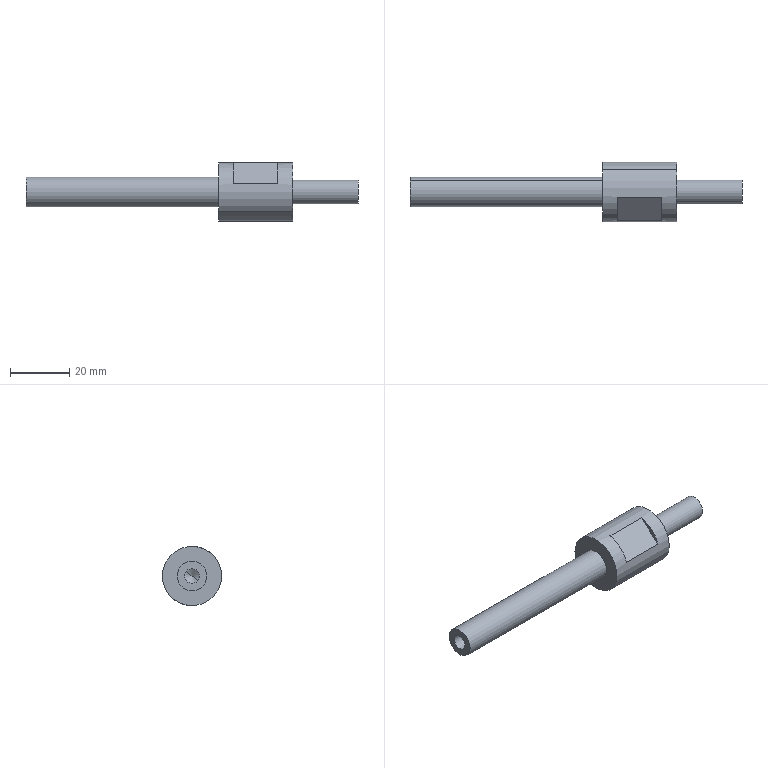Component | SolidWorks | ElectricalBoxAssembly2-1_RollerAxis-1 | 1 solid | 20 faces | box 112 x 20 x 20 mm | volume 13341 mm3 | plane 10 | cylinder 8 | cone 2 | commonest cylinder face diameters 5 x2 10 x2 20 x2 8 x2
build123d program:
from build123d import *

# Parameters (mm, degrees)
CUT_EXTRUDE1_DEPTH      = 113.889
CUT_EXTRUDE1_DEPTH_BACK = 113.889
SKETCH2_W               = 15
SKETCH2_H               = 1.5
M6_TAPPED_HOLE1_D       = 5
M6_TAPPED_HOLE1_DEPTH   = 20
M6_TAPPED_HOLE1_TIP     = 1.502


with BuildPart() as part:
    # Sketch1 → Revolve1 (revolve)
    with BuildSketch(Plane.XY, mode=Mode.PRIVATE) as revolve1_sk:
        Polygon((0, 0), (112, 0), (112, 5), (47, 5), (47, 10), (22, 10), (22, 4), (0, 4), align=None)
    revolve(revolve1_sk.sketch.rotate(Axis((0, 0, 0), (1, 0, 0)), 90), axis=Axis((0, 0, 0), (1, 0, 0)))

    # Sketch2 → Cut-Extrude1 (cut, two sides: drawn at the far end of the back side and taken through both)
    with BuildSketch(Plane.XY.offset(-CUT_EXTRUDE1_DEPTH_BACK)):
        with Locations((34.5, 9.25)):
            Rectangle(SKETCH2_W, SKETCH2_H)
        with Locations((34.5, -9.25)):
            Rectangle(SKETCH2_W, SKETCH2_H)
    extrude(amount=CUT_EXTRUDE1_DEPTH + CUT_EXTRUDE1_DEPTH_BACK, mode=Mode.SUBTRACT)

    # M6 Tapped Hole1
    with Locations(Plane(origin=(112, 0, 0), x_dir=(0, 0, -1), z_dir=(1, 0, 0))):
        with Locations((0, 0)):
            Hole(M6_TAPPED_HOLE1_D / 2, depth=M6_TAPPED_HOLE1_DEPTH)
            with Locations((0, 0, -(M6_TAPPED_HOLE1_DEPTH + M6_TAPPED_HOLE1_TIP / 2))):  # 118° drill point
                Cone(0, M6_TAPPED_HOLE1_D / 2, M6_TAPPED_HOLE1_TIP, mode=Mode.SUBTRACT)


solid = part.part

# Placed as in the assembly
solid = solid.moved(Location((765.468, -65.334, 1576.399), (-48.376, 0, 180)))
STEP:
#1=COLOUR_RGB('',0.7922,0.8196,0.9333);
#2=FILL_AREA_STYLE_COLOUR('',#1);
#3=FILL_AREA_STYLE('',(#2));
#4=SURFACE_STYLE_FILL_AREA(#3);
#5=SURFACE_SIDE_STYLE('',(#4));
#6=SURFACE_STYLE_USAGE(.BOTH.,#5);
#7=PRESENTATION_STYLE_ASSIGNMENT((#6));
#8=CARTESIAN_POINT('',(26.514,-2.499,62.128));
#9=VERTEX_POINT('',#8);
#10=CARTESIAN_POINT('',(26.514,-2.646,61.998));
#11=VERTEX_POINT('',#10);
#12=CARTESIAN_POINT('',(26.514,-2.572,62.063));
#13=DIRECTION('',(-1.,0.,-0.));
#14=DIRECTION('',(0.,-0.7475,-0.6642));
#15=AXIS2_PLACEMENT_3D('',#12,#13,#14);
#16=CIRCLE('',#15,0.09843);
#17=EDGE_CURVE('',#9,#11,#16,.T.);
#18=ORIENTED_EDGE('',*,*,#17,.F.);
#19=CARTESIAN_POINT('',(25.727,-2.499,62.128));
#20=VERTEX_POINT('',#19);
#21=CARTESIAN_POINT('',(25.727,-2.499,62.128));
#22=DIRECTION('',(-1.,0.,-0.));
#23=VECTOR('',#22,39.37);
#24=LINE('',#21,#23);
#25=EDGE_CURVE('',#9,#20,#24,.T.);
#26=ORIENTED_EDGE('',*,*,#25,.T.);
#27=CARTESIAN_POINT('',(25.727,-2.646,61.998));
#28=VERTEX_POINT('',#27);
#29=CARTESIAN_POINT('',(25.727,-2.572,62.063));
#30=DIRECTION('',(-1.,0.,-0.));
#31=DIRECTION('',(0.,-0.7475,-0.6642));
#32=AXIS2_PLACEMENT_3D('',#29,#30,#31);
#33=CIRCLE('',#32,0.09843);
#34=EDGE_CURVE('',#20,#28,#33,.T.);
#35=ORIENTED_EDGE('',*,*,#34,.T.);
#36=CARTESIAN_POINT('',(25.727,-2.646,61.998));
#37=DIRECTION('',(-1.,0.,-0.));
#38=VECTOR('',#37,39.37);
#39=LINE('',#36,#38);
#40=EDGE_CURVE('',#11,#28,#39,.T.);
#41=ORIENTED_EDGE('',*,*,#40,.F.);
#42=EDGE_LOOP('',(#18,#26,#35,#41));
#43=FACE_OUTER_BOUND('',#42,.T.);
#44=CARTESIAN_POINT('',(25.727,-2.572,62.063));
#45=DIRECTION('',(-1.,0.,-0.));
#46=DIRECTION('',(0.,-0.7475,-0.6642));
#47=AXIS2_PLACEMENT_3D('',#44,#45,#46);
#48=CYLINDRICAL_SURFACE('',#47,0.09843);
#49=ADVANCED_FACE('',(#43),#48,.F.);
#50=CARTESIAN_POINT('',(26.574,-2.572,62.063));
#51=VERTEX_POINT('',#50);
#52=CARTESIAN_POINT('',(26.514,-2.646,61.998));
#53=DIRECTION('',(-0.515,-0.6408,-0.5694));
#54=VECTOR('',#53,39.37);
#55=LINE('',#52,#54);
#56=EDGE_CURVE('',#51,#11,#55,.T.);
#57=ORIENTED_EDGE('',*,*,#56,.F.);
#58=CARTESIAN_POINT('',(26.514,-2.499,62.128));
#59=DIRECTION('',(-0.515,0.6408,0.5694));
#60=VECTOR('',#59,39.37);
#61=LINE('',#58,#60);
#62=EDGE_CURVE('',#51,#9,#61,.T.);
#63=ORIENTED_EDGE('',*,*,#62,.T.);
#64=ORIENTED_EDGE('',*,*,#17,.T.);
#65=EDGE_LOOP('',(#57,#63,#64));
#66=FACE_OUTER_BOUND('',#65,.T.);
#67=CARTESIAN_POINT('',(26.514,-2.572,62.063));
#68=DIRECTION('',(-1.,0.,-0.));
#69=DIRECTION('',(0.,-0.7475,-0.6642));
#70=AXIS2_PLACEMENT_3D('',#67,#68,#69);
#71=CONICAL_SURFACE('',#70,0.09843,1.03);
#72=ADVANCED_FACE('',(#66),#71,.F.);
#73=CARTESIAN_POINT('',(25.727,-2.425,62.194));
#74=VERTEX_POINT('',#73);
#75=CARTESIAN_POINT('',(25.727,-2.719,61.932));
#76=VERTEX_POINT('',#75);
#77=CARTESIAN_POINT('',(25.727,-2.572,62.063));
#78=DIRECTION('',(1.,-0.,0.));
#79=DIRECTION('',(0.,0.7475,0.6642));
#80=AXIS2_PLACEMENT_3D('',#77,#78,#79);
#81=CIRCLE('',#80,0.1969);
#82=EDGE_CURVE('',#74,#76,#81,.T.);
#83=ORIENTED_EDGE('',*,*,#82,.T.);
#84=CARTESIAN_POINT('',(28.286,-2.719,61.932));
#85=VERTEX_POINT('',#84);
#86=CARTESIAN_POINT('',(30.137,-2.719,61.932));
#87=DIRECTION('',(1.,-0.,0.));
#88=VECTOR('',#87,39.37);
#89=LINE('',#86,#88);
#90=EDGE_CURVE('',#76,#85,#89,.T.);
#91=ORIENTED_EDGE('',*,*,#90,.T.);
#92=CARTESIAN_POINT('',(28.286,-2.425,62.194));
#93=VERTEX_POINT('',#92);
#94=CARTESIAN_POINT('',(28.286,-2.572,62.063));
#95=DIRECTION('',(1.,-0.,0.));
#96=DIRECTION('',(0.,0.7475,0.6642));
#97=AXIS2_PLACEMENT_3D('',#94,#95,#96);
#98=CIRCLE('',#97,0.1969);
#99=EDGE_CURVE('',#93,#85,#98,.T.);
#100=ORIENTED_EDGE('',*,*,#99,.F.);
#101=CARTESIAN_POINT('',(30.137,-2.425,62.194));
#102=DIRECTION('',(1.,-0.,0.));
#103=VECTOR('',#102,39.37);
#104=LINE('',#101,#103);
#105=EDGE_CURVE('',#74,#93,#104,.T.);
#106=ORIENTED_EDGE('',*,*,#105,.F.);
#107=EDGE_LOOP('',(#83,#91,#100,#106));
#108=FACE_OUTER_BOUND('',#107,.T.);
#109=CARTESIAN_POINT('',(30.137,-2.572,62.063));
#110=DIRECTION('',(1.,-0.,0.));
#111=DIRECTION('',(0.,0.7475,0.6642));
#112=AXIS2_PLACEMENT_3D('',#109,#110,#111);
#113=CYLINDRICAL_SURFACE('',#112,0.1969);
#114=ADVANCED_FACE('',(#108),#113,.T.);
#115=CARTESIAN_POINT('',(28.483,-2.95,62.175));
#116=VERTEX_POINT('',#115);
#117=CARTESIAN_POINT('',(28.483,-2.639,62.451));
#118=VERTEX_POINT('',#117);
#119=CARTESIAN_POINT('',(28.483,-2.572,62.063));
#120=DIRECTION('',(-1.,-0.,0.));
#121=DIRECTION('',(0.,-0.6642,0.7475));
#122=AXIS2_PLACEMENT_3D('',#119,#120,#121);
#123=CIRCLE('',#122,0.3937);
#124=EDGE_CURVE('',#116,#118,#123,.T.);
#125=ORIENTED_EDGE('',*,*,#124,.T.);
#126=CARTESIAN_POINT('',(29.074,-2.639,62.451));
#127=VERTEX_POINT('',#126);
#128=CARTESIAN_POINT('',(30.137,-2.639,62.451));
#129=DIRECTION('',(1.,-0.,0.));
#130=VECTOR('',#129,39.37);
#131=LINE('',#128,#130);
#132=EDGE_CURVE('',#118,#127,#131,.T.);
#133=ORIENTED_EDGE('',*,*,#132,.T.);
#134=CARTESIAN_POINT('',(29.074,-2.95,62.175));
#135=VERTEX_POINT('',#134);
#136=CARTESIAN_POINT('',(29.074,-2.572,62.063));
#137=DIRECTION('',(1.,-0.,0.));
#138=DIRECTION('',(0.,0.7475,0.6642));
#139=AXIS2_PLACEMENT_3D('',#136,#137,#138);
#140=CIRCLE('',#139,0.3937);
#141=EDGE_CURVE('',#127,#135,#140,.T.);
#142=ORIENTED_EDGE('',*,*,#141,.T.);
#143=CARTESIAN_POINT('',(30.137,-2.95,62.175));
#144=DIRECTION('',(-1.,0.,-0.));
#145=VECTOR('',#144,39.37);
#146=LINE('',#143,#145);
#147=EDGE_CURVE('',#135,#116,#146,.T.);
#148=ORIENTED_EDGE('',*,*,#147,.T.);
#149=EDGE_LOOP('',(#125,#133,#142,#148));
#150=FACE_BOUND('',#149,.T.);
#151=CARTESIAN_POINT('',(28.286,-2.278,62.324));
#152=VERTEX_POINT('',#151);
#153=CARTESIAN_POINT('',(28.286,-2.867,61.801));
#154=VERTEX_POINT('',#153);
#155=CARTESIAN_POINT('',(28.286,-2.572,62.063));
#156=DIRECTION('',(1.,-0.,0.));
#157=DIRECTION('',(0.,0.7475,0.6642));
#158=AXIS2_PLACEMENT_3D('',#155,#156,#157);
#159=CIRCLE('',#158,0.3937);
#160=EDGE_CURVE('',#152,#154,#159,.T.);
#161=ORIENTED_EDGE('',*,*,#160,.T.);
#162=CARTESIAN_POINT('',(29.27,-2.867,61.801));
#163=VERTEX_POINT('',#162);
#164=CARTESIAN_POINT('',(30.137,-2.867,61.801));
#165=DIRECTION('',(1.,-0.,0.));
#166=VECTOR('',#165,39.37);
#167=LINE('',#164,#166);
#168=EDGE_CURVE('',#154,#163,#167,.T.);
#169=ORIENTED_EDGE('',*,*,#168,.T.);
#170=CARTESIAN_POINT('',(29.27,-2.278,62.324));
#171=VERTEX_POINT('',#170);
#172=CARTESIAN_POINT('',(29.27,-2.572,62.063));
#173=DIRECTION('',(1.,-0.,0.));
#174=DIRECTION('',(0.,0.7475,0.6642));
#175=AXIS2_PLACEMENT_3D('',#172,#173,#174);
#176=CIRCLE('',#175,0.3937);
#177=EDGE_CURVE('',#171,#163,#176,.T.);
#178=ORIENTED_EDGE('',*,*,#177,.F.);
#179=CARTESIAN_POINT('',(30.137,-2.278,62.324));
#180=DIRECTION('',(1.,-0.,0.));
#181=VECTOR('',#180,39.37);
#182=LINE('',#179,#181);
#183=EDGE_CURVE('',#152,#171,#182,.T.);
#184=ORIENTED_EDGE('',*,*,#183,.F.);
#185=EDGE_LOOP('',(#161,#169,#178,#184));
#186=FACE_OUTER_BOUND('',#185,.T.);
#187=CARTESIAN_POINT('',(30.137,-2.572,62.063));
#188=DIRECTION('',(1.,-0.,0.));
#189=DIRECTION('',(0.,0.7475,0.6642));
#190=AXIS2_PLACEMENT_3D('',#187,#188,#189);
#191=CYLINDRICAL_SURFACE('',#190,0.3937);
#192=ADVANCED_FACE('',(#150,#186),#191,.T.);
#193=CARTESIAN_POINT('',(29.27,-2.454,62.168));
#194=VERTEX_POINT('',#193);
#195=CARTESIAN_POINT('',(29.27,-2.69,61.958));
#196=VERTEX_POINT('',#195);
#197=CARTESIAN_POINT('',(29.27,-2.572,62.063));
#198=DIRECTION('',(1.,-0.,0.));
#199=DIRECTION('',(0.,0.7475,0.6642));
#200=AXIS2_PLACEMENT_3D('',#197,#198,#199);
#201=CIRCLE('',#200,0.1575);
#202=EDGE_CURVE('',#194,#196,#201,.T.);
#203=ORIENTED_EDGE('',*,*,#202,.T.);
#204=CARTESIAN_POINT('',(30.137,-2.69,61.958));
#205=VERTEX_POINT('',#204);
#206=CARTESIAN_POINT('',(30.137,-2.69,61.958));
#207=DIRECTION('',(1.,-0.,0.));
#208=VECTOR('',#207,39.37);
#209=LINE('',#206,#208);
#210=EDGE_CURVE('',#196,#205,#209,.T.);
#211=ORIENTED_EDGE('',*,*,#210,.T.);
#212=CARTESIAN_POINT('',(30.137,-2.454,62.168));
#213=VERTEX_POINT('',#212);
#214=CARTESIAN_POINT('',(30.137,-2.572,62.063));
#215=DIRECTION('',(1.,-0.,0.));
#216=DIRECTION('',(0.,0.7475,0.6642));
#217=AXIS2_PLACEMENT_3D('',#214,#215,#216);
#218=CIRCLE('',#217,0.1575);
#219=EDGE_CURVE('',#213,#205,#218,.T.);
#220=ORIENTED_EDGE('',*,*,#219,.F.);
#221=CARTESIAN_POINT('',(30.137,-2.454,62.168));
#222=DIRECTION('',(1.,-0.,0.));
#223=VECTOR('',#222,39.37);
#224=LINE('',#221,#223);
#225=EDGE_CURVE('',#194,#213,#224,.T.);
#226=ORIENTED_EDGE('',*,*,#225,.F.);
#227=EDGE_LOOP('',(#203,#211,#220,#226));
#228=FACE_OUTER_BOUND('',#227,.T.);
#229=CARTESIAN_POINT('',(30.137,-2.572,62.063));
#230=DIRECTION('',(1.,-0.,0.));
#231=DIRECTION('',(0.,0.7475,0.6642));
#232=AXIS2_PLACEMENT_3D('',#229,#230,#231);
#233=CYLINDRICAL_SURFACE('',#232,0.1575);
#234=ADVANCED_FACE('',(#228),#233,.T.);
#235=ORIENTED_EDGE('',*,*,#219,.T.);
#236=CARTESIAN_POINT('',(30.137,-2.572,62.063));
#237=DIRECTION('',(1.,-0.,0.));
#238=DIRECTION('',(0.,0.7475,0.6642));
#239=AXIS2_PLACEMENT_3D('',#236,#237,#238);
#240=CIRCLE('',#239,0.1575);
#241=EDGE_CURVE('',#205,#213,#240,.T.);
#242=ORIENTED_EDGE('',*,*,#241,.T.);
#243=EDGE_LOOP('',(#235,#242));
#244=FACE_OUTER_BOUND('',#243,.T.);
#245=CARTESIAN_POINT('',(30.137,-2.572,62.063));
#246=DIRECTION('',(-1.,-0.,-0.));
#247=DIRECTION('',(0.,-0.7475,-0.6642));
#248=AXIS2_PLACEMENT_3D('',#245,#246,#247);
#249=PLANE('',#248);
#250=ADVANCED_FACE('',(#244),#249,.F.);
#251=ORIENTED_EDGE('',*,*,#210,.F.);
#252=CARTESIAN_POINT('',(29.27,-2.572,62.063));
#253=DIRECTION('',(1.,-0.,0.));
#254=DIRECTION('',(0.,0.7475,0.6642));
#255=AXIS2_PLACEMENT_3D('',#252,#253,#254);
#256=CIRCLE('',#255,0.1575);
#257=EDGE_CURVE('',#196,#194,#256,.T.);
#258=ORIENTED_EDGE('',*,*,#257,.T.);
#259=ORIENTED_EDGE('',*,*,#225,.T.);
#260=ORIENTED_EDGE('',*,*,#241,.F.);
#261=EDGE_LOOP('',(#251,#258,#259,#260));
#262=FACE_OUTER_BOUND('',#261,.T.);
#263=CARTESIAN_POINT('',(30.137,-2.572,62.063));
#264=DIRECTION('',(1.,-0.,0.));
#265=DIRECTION('',(0.,0.7475,0.6642));
#266=AXIS2_PLACEMENT_3D('',#263,#264,#265);
#267=CYLINDRICAL_SURFACE('',#266,0.1575);
#268=ADVANCED_FACE('',(#262),#267,.T.);
#269=ORIENTED_EDGE('',*,*,#202,.F.);
#270=ORIENTED_EDGE('',*,*,#257,.F.);
#271=EDGE_LOOP('',(#269,#270));
#272=FACE_BOUND('',#271,.T.);
#273=ORIENTED_EDGE('',*,*,#177,.T.);
#274=CARTESIAN_POINT('',(29.27,-2.572,62.063));
#275=DIRECTION('',(1.,-0.,0.));
#276=DIRECTION('',(0.,0.7475,0.6642));
#277=AXIS2_PLACEMENT_3D('',#274,#275,#276);
#278=CIRCLE('',#277,0.3937);
#279=EDGE_CURVE('',#163,#171,#278,.T.);
#280=ORIENTED_EDGE('',*,*,#279,.T.);
#281=EDGE_LOOP('',(#273,#280));
#282=FACE_OUTER_BOUND('',#281,.T.);
#283=CARTESIAN_POINT('',(29.27,-2.677,62.181));
#284=DIRECTION('',(-1.,-0.,-0.));
#285=DIRECTION('',(0.,-0.7475,-0.6642));
#286=AXIS2_PLACEMENT_3D('',#283,#284,#285);
#287=PLANE('',#286);
#288=ADVANCED_FACE('',(#272,#282),#287,.F.);
#289=ORIENTED_EDGE('',*,*,#168,.F.);
#290=CARTESIAN_POINT('',(28.286,-2.572,62.063));
#291=DIRECTION('',(1.,-0.,0.));
#292=DIRECTION('',(0.,0.7475,0.6642));
#293=AXIS2_PLACEMENT_3D('',#290,#291,#292);
#294=CIRCLE('',#293,0.3937);
#295=EDGE_CURVE('',#154,#152,#294,.T.);
#296=ORIENTED_EDGE('',*,*,#295,.T.);
#297=ORIENTED_EDGE('',*,*,#183,.T.);
#298=ORIENTED_EDGE('',*,*,#279,.F.);
#299=EDGE_LOOP('',(#289,#296,#297,#298));
#300=FACE_OUTER_BOUND('',#299,.T.);
#301=CARTESIAN_POINT('',(28.483,-2.505,61.675));
#302=VERTEX_POINT('',#301);
#303=CARTESIAN_POINT('',(29.074,-2.505,61.675));
#304=VERTEX_POINT('',#303);
#305=CARTESIAN_POINT('',(30.137,-2.505,61.675));
#306=DIRECTION('',(1.,-0.,0.));
#307=VECTOR('',#306,39.37);
#308=LINE('',#305,#307);
#309=EDGE_CURVE('',#302,#304,#308,.T.);
#310=ORIENTED_EDGE('',*,*,#309,.T.);
#311=CARTESIAN_POINT('',(29.074,-2.195,61.951));
#312=VERTEX_POINT('',#311);
#313=CARTESIAN_POINT('',(29.074,-2.572,62.063));
#314=DIRECTION('',(1.,-0.,0.));
#315=DIRECTION('',(0.,0.7475,0.6642));
#316=AXIS2_PLACEMENT_3D('',#313,#314,#315);
#317=CIRCLE('',#316,0.3937);
#318=EDGE_CURVE('',#304,#312,#317,.T.);
#319=ORIENTED_EDGE('',*,*,#318,.T.);
#320=CARTESIAN_POINT('',(28.483,-2.195,61.951));
#321=VERTEX_POINT('',#320);
#322=CARTESIAN_POINT('',(30.137,-2.195,61.951));
#323=DIRECTION('',(-1.,0.,-0.));
#324=VECTOR('',#323,39.37);
#325=LINE('',#322,#324);
#326=EDGE_CURVE('',#312,#321,#325,.T.);
#327=ORIENTED_EDGE('',*,*,#326,.T.);
#328=CARTESIAN_POINT('',(28.483,-2.572,62.063));
#329=DIRECTION('',(-1.,0.,-0.));
#330=DIRECTION('',(0.,-0.6642,0.7475));
#331=AXIS2_PLACEMENT_3D('',#328,#329,#330);
#332=CIRCLE('',#331,0.3937);
#333=EDGE_CURVE('',#321,#302,#332,.T.);
#334=ORIENTED_EDGE('',*,*,#333,.T.);
#335=EDGE_LOOP('',(#310,#319,#327,#334));
#336=FACE_BOUND('',#335,.T.);
#337=CARTESIAN_POINT('',(30.137,-2.572,62.063));
#338=DIRECTION('',(1.,-0.,0.));
#339=DIRECTION('',(0.,0.7475,0.6642));
#340=AXIS2_PLACEMENT_3D('',#337,#338,#339);
#341=CYLINDRICAL_SURFACE('',#340,0.3937);
#342=ADVANCED_FACE('',(#300,#336),#341,.T.);
#343=ORIENTED_EDGE('',*,*,#160,.F.);
#344=ORIENTED_EDGE('',*,*,#295,.F.);
#345=EDGE_LOOP('',(#343,#344));
#346=FACE_OUTER_BOUND('',#345,.T.);
#347=ORIENTED_EDGE('',*,*,#99,.T.);
#348=CARTESIAN_POINT('',(28.286,-2.572,62.063));
#349=DIRECTION('',(1.,-0.,0.));
#350=DIRECTION('',(0.,0.7475,0.6642));
#351=AXIS2_PLACEMENT_3D('',#348,#349,#350);
#352=CIRCLE('',#351,0.1969);
#353=EDGE_CURVE('',#85,#93,#352,.T.);
#354=ORIENTED_EDGE('',*,*,#353,.T.);
#355=EDGE_LOOP('',(#347,#354));
#356=FACE_BOUND('',#355,.T.);
#357=CARTESIAN_POINT('',(28.286,-2.834,62.357));
#358=DIRECTION('',(1.,0.,0.));
#359=DIRECTION('',(-0.,0.7475,0.6642));
#360=AXIS2_PLACEMENT_3D('',#357,#358,#359);
#361=PLANE('',#360);
#362=ADVANCED_FACE('',(#346,#356),#361,.F.);
#363=ORIENTED_EDGE('',*,*,#90,.F.);
#364=CARTESIAN_POINT('',(25.727,-2.572,62.063));
#365=DIRECTION('',(1.,-0.,0.));
#366=DIRECTION('',(0.,0.7475,0.6642));
#367=AXIS2_PLACEMENT_3D('',#364,#365,#366);
#368=CIRCLE('',#367,0.1969);
#369=EDGE_CURVE('',#76,#74,#368,.T.);
#370=ORIENTED_EDGE('',*,*,#369,.T.);
#371=ORIENTED_EDGE('',*,*,#105,.T.);
#372=ORIENTED_EDGE('',*,*,#353,.F.);
#373=EDGE_LOOP('',(#363,#370,#371,#372));
#374=FACE_OUTER_BOUND('',#373,.T.);
#375=CARTESIAN_POINT('',(30.137,-2.572,62.063));
#376=DIRECTION('',(1.,-0.,0.));
#377=DIRECTION('',(0.,0.7475,0.6642));
#378=AXIS2_PLACEMENT_3D('',#375,#376,#377);
#379=CYLINDRICAL_SURFACE('',#378,0.1969);
#380=ADVANCED_FACE('',(#374),#379,.T.);
#381=CARTESIAN_POINT('',(25.727,-2.572,62.063));
#382=DIRECTION('',(-1.,0.,-0.));
#383=DIRECTION('',(0.,-0.7475,-0.6642));
#384=AXIS2_PLACEMENT_3D('',#381,#382,#383);
#385=CIRCLE('',#384,0.09843);
#386=EDGE_CURVE('',#28,#20,#385,.T.);
#387=ORIENTED_EDGE('',*,*,#386,.F.);
#388=ORIENTED_EDGE('',*,*,#34,.F.);
#389=EDGE_LOOP('',(#387,#388));
#390=FACE_BOUND('',#389,.T.);
#391=ORIENTED_EDGE('',*,*,#82,.F.);
#392=ORIENTED_EDGE('',*,*,#369,.F.);
#393=EDGE_LOOP('',(#391,#392));
#394=FACE_OUTER_BOUND('',#393,.T.);
#395=CARTESIAN_POINT('',(25.727,-2.703,62.21));
#396=DIRECTION('',(1.,0.,0.));
#397=DIRECTION('',(-0.,0.7475,0.6642));
#398=AXIS2_PLACEMENT_3D('',#395,#396,#397);
#399=PLANE('',#398);
#400=ADVANCED_FACE('',(#390,#394),#399,.F.);
#401=CARTESIAN_POINT('',(29.074,-3.089,62.052));
#402=DIRECTION('',(-0.,0.7475,0.6642));
#403=VECTOR('',#402,39.37);
#404=LINE('',#401,#403);
#405=EDGE_CURVE('',#135,#127,#404,.T.);
#406=ORIENTED_EDGE('',*,*,#405,.F.);
#407=ORIENTED_EDGE('',*,*,#141,.F.);
#408=EDGE_LOOP('',(#406,#407));
#409=FACE_OUTER_BOUND('',#408,.T.);
#410=CARTESIAN_POINT('',(29.074,-3.128,62.096));
#411=DIRECTION('',(1.,0.,0.));
#412=DIRECTION('',(-0.,0.7475,0.6642));
#413=AXIS2_PLACEMENT_3D('',#410,#411,#412);
#414=PLANE('',#413);
#415=ADVANCED_FACE('',(#409),#414,.F.);
#416=ORIENTED_EDGE('',*,*,#124,.F.);
#417=CARTESIAN_POINT('',(28.483,-3.089,62.052));
#418=DIRECTION('',(-0.,0.7475,0.6642));
#419=VECTOR('',#418,39.37);
#420=LINE('',#417,#419);
#421=EDGE_CURVE('',#116,#118,#420,.T.);
#422=ORIENTED_EDGE('',*,*,#421,.T.);
#423=EDGE_LOOP('',(#416,#422));
#424=FACE_OUTER_BOUND('',#423,.T.);
#425=CARTESIAN_POINT('',(28.483,-3.128,62.096));
#426=DIRECTION('',(-1.,-0.,0.));
#427=DIRECTION('',(0.,-0.6642,0.7475));
#428=AXIS2_PLACEMENT_3D('',#425,#426,#427);
#429=PLANE('',#428);
#430=ADVANCED_FACE('',(#424),#429,.F.);
#431=ORIENTED_EDGE('',*,*,#421,.F.);
#432=ORIENTED_EDGE('',*,*,#147,.F.);
#433=ORIENTED_EDGE('',*,*,#405,.T.);
#434=ORIENTED_EDGE('',*,*,#132,.F.);
#435=EDGE_LOOP('',(#431,#432,#433,#434));
#436=FACE_OUTER_BOUND('',#435,.T.);
#437=CARTESIAN_POINT('',(29.074,-3.089,62.052));
#438=DIRECTION('',(0.,0.6642,-0.7475));
#439=DIRECTION('',(0.,-0.7475,-0.6642));
#440=AXIS2_PLACEMENT_3D('',#437,#438,#439);
#441=PLANE('',#440);
#442=ADVANCED_FACE('',(#436),#441,.F.);
#443=CARTESIAN_POINT('',(29.074,-2.644,61.551));
#444=DIRECTION('',(-0.,0.7475,0.6642));
#445=VECTOR('',#444,39.37);
#446=LINE('',#443,#445);
#447=EDGE_CURVE('',#304,#312,#446,.T.);
#448=ORIENTED_EDGE('',*,*,#447,.T.);
#449=ORIENTED_EDGE('',*,*,#318,.F.);
#450=EDGE_LOOP('',(#448,#449));
#451=FACE_OUTER_BOUND('',#450,.T.);
#452=CARTESIAN_POINT('',(29.074,-2.605,61.507));
#453=DIRECTION('',(1.,0.,0.));
#454=DIRECTION('',(-0.,0.7475,0.6642));
#455=AXIS2_PLACEMENT_3D('',#452,#453,#454);
#456=PLANE('',#455);
#457=ADVANCED_FACE('',(#451),#456,.F.);
#458=CARTESIAN_POINT('',(28.483,-2.644,61.551));
#459=DIRECTION('',(-0.,0.7475,0.6642));
#460=VECTOR('',#459,39.37);
#461=LINE('',#458,#460);
#462=EDGE_CURVE('',#302,#321,#461,.T.);
#463=ORIENTED_EDGE('',*,*,#462,.T.);
#464=ORIENTED_EDGE('',*,*,#326,.F.);
#465=ORIENTED_EDGE('',*,*,#447,.F.);
#466=ORIENTED_EDGE('',*,*,#309,.F.);
#467=EDGE_LOOP('',(#463,#464,#465,#466));
#468=FACE_OUTER_BOUND('',#467,.T.);
#469=CARTESIAN_POINT('',(29.074,-2.644,61.551));
#470=DIRECTION('',(-0.,-0.6642,0.7475));
#471=DIRECTION('',(-0.,0.7475,0.6642));
#472=AXIS2_PLACEMENT_3D('',#469,#470,#471);
#473=PLANE('',#472);
#474=ADVANCED_FACE('',(#468),#473,.F.);
#475=ORIENTED_EDGE('',*,*,#462,.F.);
#476=ORIENTED_EDGE('',*,*,#333,.F.);
#477=EDGE_LOOP('',(#475,#476));
#478=FACE_OUTER_BOUND('',#477,.T.);
#479=CARTESIAN_POINT('',(28.483,-2.605,61.507));
#480=DIRECTION('',(-1.,0.,-0.));
#481=DIRECTION('',(-0.,-0.6642,0.7475));
#482=AXIS2_PLACEMENT_3D('',#479,#480,#481);
#483=PLANE('',#482);
#484=ADVANCED_FACE('',(#478),#483,.F.);
#485=ORIENTED_EDGE('',*,*,#62,.F.);
#486=ORIENTED_EDGE('',*,*,#56,.T.);
#487=CARTESIAN_POINT('',(26.514,-2.572,62.063));
#488=DIRECTION('',(-1.,0.,-0.));
#489=DIRECTION('',(0.,-0.7475,-0.6642));
#490=AXIS2_PLACEMENT_3D('',#487,#488,#489);
#491=CIRCLE('',#490,0.09843);
#492=EDGE_CURVE('',#11,#9,#491,.T.);
#493=ORIENTED_EDGE('',*,*,#492,.T.);
#494=EDGE_LOOP('',(#485,#486,#493));
#495=FACE_OUTER_BOUND('',#494,.T.);
#496=CARTESIAN_POINT('',(26.514,-2.572,62.063));
#497=DIRECTION('',(-1.,0.,-0.));
#498=DIRECTION('',(0.,-0.7475,-0.6642));
#499=AXIS2_PLACEMENT_3D('',#496,#497,#498);
#500=CONICAL_SURFACE('',#499,0.09843,1.03);
#501=ADVANCED_FACE('',(#495),#500,.F.);
#502=ORIENTED_EDGE('',*,*,#25,.F.);
#503=ORIENTED_EDGE('',*,*,#492,.F.);
#504=ORIENTED_EDGE('',*,*,#40,.T.);
#505=ORIENTED_EDGE('',*,*,#386,.T.);
#506=EDGE_LOOP('',(#502,#503,#504,#505));
#507=FACE_OUTER_BOUND('',#506,.T.);
#508=CARTESIAN_POINT('',(25.727,-2.572,62.063));
#509=DIRECTION('',(-1.,0.,-0.));
#510=DIRECTION('',(0.,-0.7475,-0.6642));
#511=AXIS2_PLACEMENT_3D('',#508,#509,#510);
#512=CYLINDRICAL_SURFACE('',#511,0.09843);
#513=ADVANCED_FACE('',(#507),#512,.F.);
#514=CLOSED_SHELL('',(#49,#72,#114,#192,#234,#250,#268,#288,#342,#362,#380,#400,#415,#430,#442,#457,#474,#484,#501,#513));
#515=MANIFOLD_SOLID_BREP('',#514);
#516=STYLED_ITEM('',(#7),#515);
#517=PRESENTATION_LAYER_ASSIGNMENT('','',(#516));
#518=CARTESIAN_POINT('',(0.,0.,0.));
#519=DIRECTION('',(0.,0.,1.));
#520=DIRECTION('',(1.,0.,0.));
#521=AXIS2_PLACEMENT_3D('',#518,#519,#520);
#522=(LENGTH_UNIT()NAMED_UNIT(*)SI_UNIT($,.METRE.));
#523=LENGTH_MEASURE_WITH_UNIT(LENGTH_MEASURE(0.0254),#522);
#524=DIMENSIONAL_EXPONENTS(1.,0.,0.,0.,0.,0.,0.);
#525=(CONVERSION_BASED_UNIT('',#523)LENGTH_UNIT()NAMED_UNIT(#524));
#526=UNCERTAINTY_MEASURE_WITH_UNIT(LENGTH_MEASURE(0.00001),#525,'','');
#527=(NAMED_UNIT(*)PLANE_ANGLE_UNIT()SI_UNIT($,.RADIAN.));
#528=(NAMED_UNIT(*)SI_UNIT($,.STERADIAN.)SOLID_ANGLE_UNIT());
#529=(GEOMETRIC_REPRESENTATION_CONTEXT(3)GLOBAL_UNCERTAINTY_ASSIGNED_CONTEXT((#526))GLOBAL_UNIT_ASSIGNED_CONTEXT((#525,#527,#528))REPRESENTATION_CONTEXT('',''));
#530=ADVANCED_BREP_SHAPE_REPRESENTATION('',(#515,#521),#529);
#531=(LENGTH_UNIT()NAMED_UNIT(*)SI_UNIT($,.METRE.));
#532=LENGTH_MEASURE_WITH_UNIT(LENGTH_MEASURE(0.0254),#531);
#533=DIMENSIONAL_EXPONENTS(1.,0.,0.,0.,0.,0.,0.);
#534=(CONVERSION_BASED_UNIT('',#532)LENGTH_UNIT()NAMED_UNIT(#533));
#535=UNCERTAINTY_MEASURE_WITH_UNIT(LENGTH_MEASURE(0.00001),#534,'','');
#536=(NAMED_UNIT(*)PLANE_ANGLE_UNIT()SI_UNIT($,.RADIAN.));
#537=(NAMED_UNIT(*)SI_UNIT($,.STERADIAN.)SOLID_ANGLE_UNIT());
#538=(GEOMETRIC_REPRESENTATION_CONTEXT(3)GLOBAL_UNCERTAINTY_ASSIGNED_CONTEXT((#535))GLOBAL_UNIT_ASSIGNED_CONTEXT((#534,#536,#537))REPRESENTATION_CONTEXT('',''));
#539=MECHANICAL_DESIGN_GEOMETRIC_PRESENTATION_REPRESENTATION('',(#516),#538);